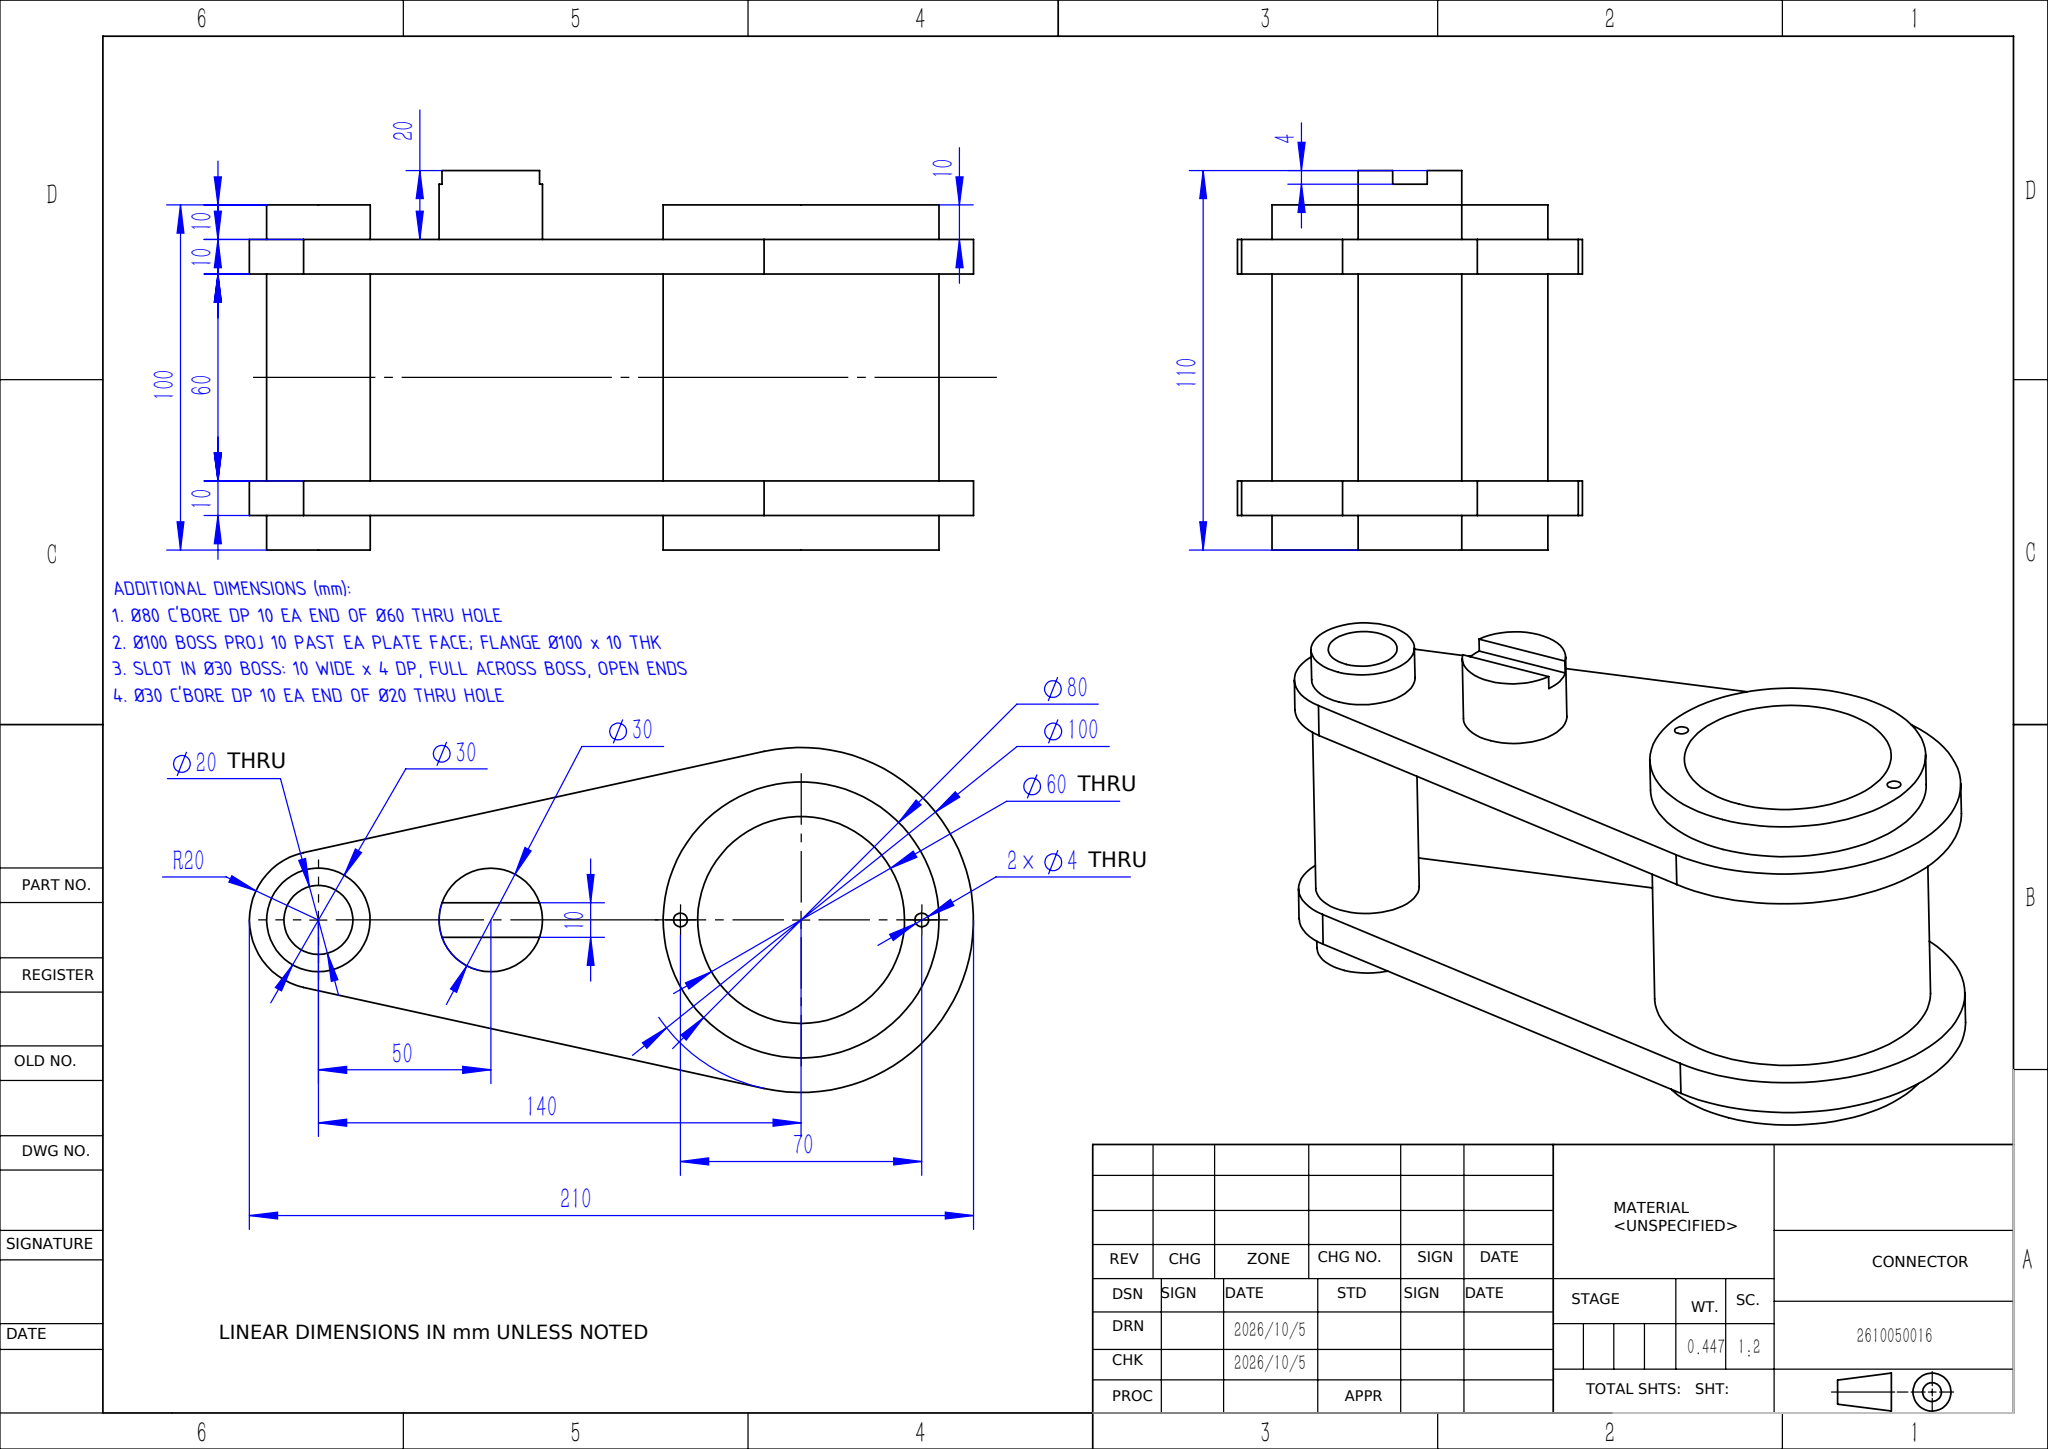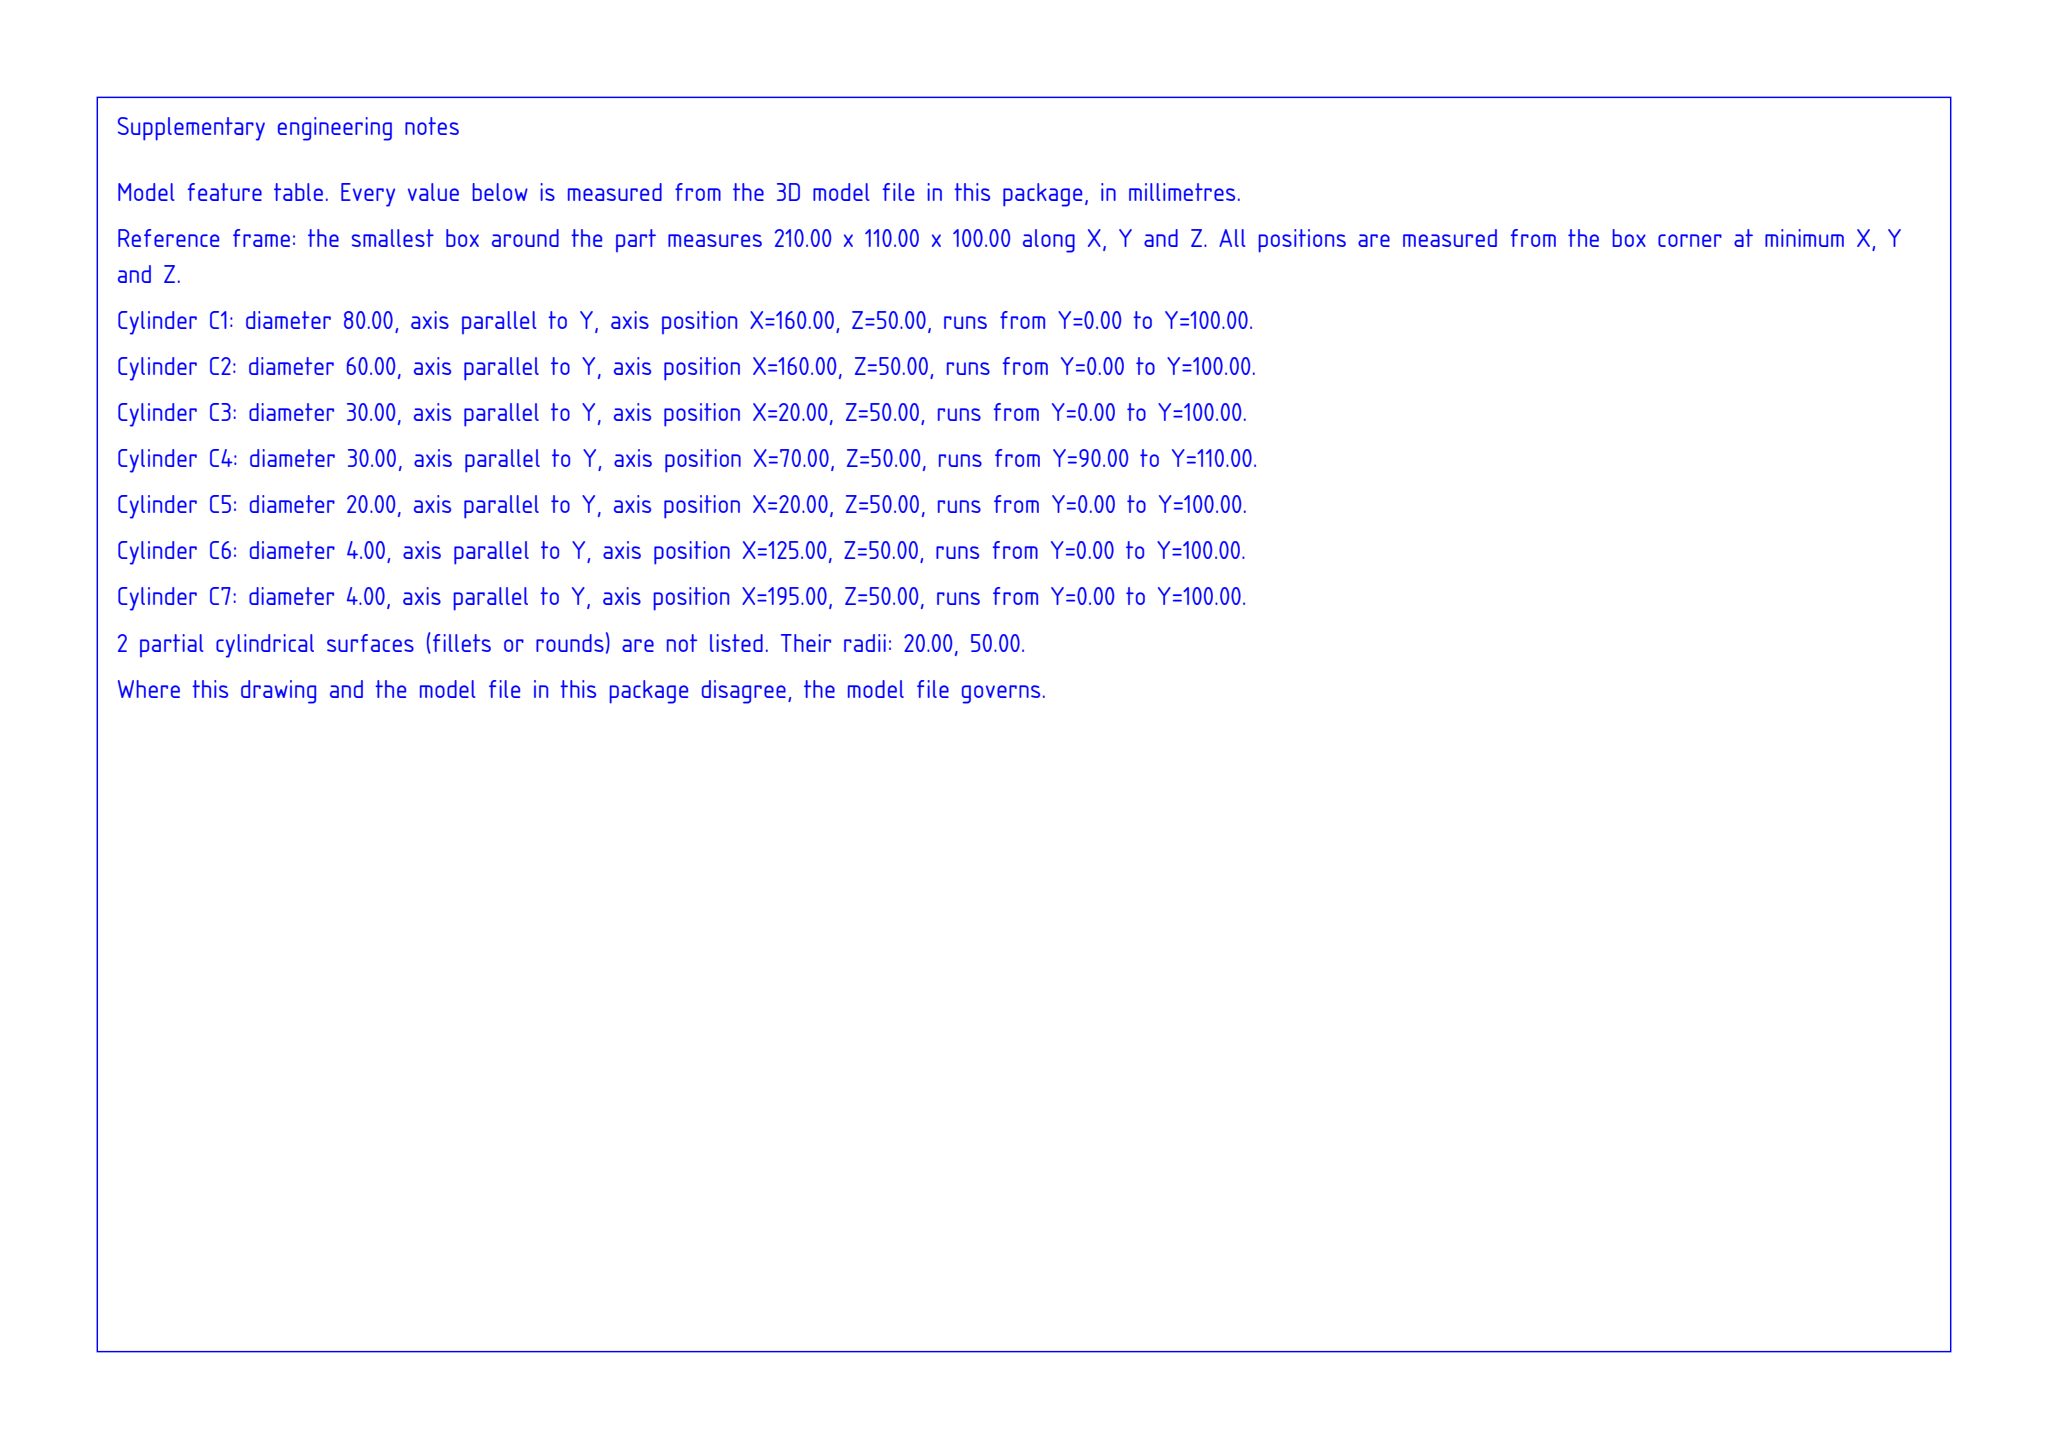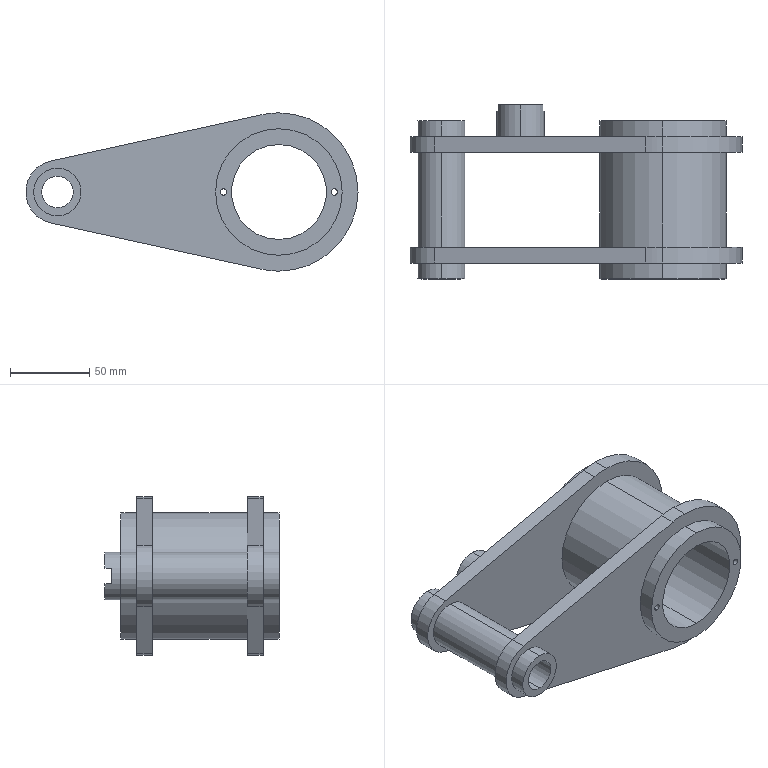Part | SolidWorks | mm | 1 solid | 47 faces | box 210 x 110 x 100 mm | volume 446583 mm3 | cylinder 30 | plane 17 | commonest cylinder face diameters 30 x8 80 x6 100 x6 4 x4 20 x2 60 x2 40 x2
build123d program:
from build123d import *

# Parameters (mm, degrees)
BOSS_EXTRUDE1_DEPTH     = 40
CUT_EXTRUDE1_DEPTH      = 137.015
CUT_EXTRUDE1_DEPTH_BACK = 137.015
SKETCH2_W               = 210
SKETCH2_H               = 60
SKETCH3_R               = 15
SKETCH3_R_2             = 40
BOSS_EXTRUDE2_DEPTH     = 50
CUT_EXTRUDE2_DEPTH      = 165.012
CUT_EXTRUDE2_DEPTH_BACK = 165.012
SKETCH4_R               = 10
SKETCH4_R_2             = 30
SKETCH5_R               = 15
BOSS_EXTRUDE3_DEPTH     = 20
CUT_EXTRUDE3_DEPTH      = 171.294
CUT_EXTRUDE3_DEPTH_BACK = 4
SKETCH6_W               = 33.027
SKETCH6_H               = 10
SKETCH7_R               = 2
CUT_EXTRUDE4_DEPTH      = 165.012


with BuildPart() as part:
    # Sketch1 → Boss-Extrude1 (new, symmetric)
    with BuildSketch(Plane(origin=(0, 0, 0), x_dir=(1, 0, 0), z_dir=(0, 1, 0))):
        with BuildLine():
            Line((-74.286, 19.535), (59.286, 48.839))
            ThreePointArc((59.286, 48.839), (120, 0), (59.286, -48.839))
            Line((59.286, -48.839), (-74.286, -19.535))
            ThreePointArc((-74.286, -19.535), (-90, 0), (-74.286, 19.535))
        make_face()
    extrude(amount=BOSS_EXTRUDE1_DEPTH, both=True)

    # Sketch2 → Cut-Extrude1 (cut, two sides: drawn at the far end of the back side and taken through both)
    with BuildSketch(Plane.XY.offset(-CUT_EXTRUDE1_DEPTH_BACK)):
        with Locations((15, 0)):
            Rectangle(SKETCH2_W, SKETCH2_H)
    extrude(amount=CUT_EXTRUDE1_DEPTH + CUT_EXTRUDE1_DEPTH_BACK, mode=Mode.SUBTRACT)


with BuildPart() as cut_extrude1_piece_1:
    # of the separate pieces the step leaves, piece 1, a body of its own (cut_extrude1_pieces)
    add(part.part.solids().sort_by_distance((59.286, 30, 48.839))[0])



with BuildPart() as cut_extrude1_piece_2:
    # of the separate pieces the step leaves, piece 2, a body of its own (cut_extrude1_pieces)
    add(part.part.solids().sort_by_distance((59.286, -40, 48.839))[0])


with BuildPart() as cut_extrude1_piece_1_1:
    add(cut_extrude1_piece_1.part)

    add(cut_extrude1_piece_2.part)  # Boss-Extrude2 merges Cut-Extrude1 piece 2
    # Sketch3 → Boss-Extrude2 (add, symmetric)
    with BuildSketch(Plane(origin=(0, 0, 0), x_dir=(1, 0, 0), z_dir=(0, 1, 0))):
        with Locations(Location((-70, 0, 0), (0, 0, 90))):
            Circle(SKETCH3_R)
        with Locations(Location((70, 0, 0), (0, 0, 90))):
            Circle(SKETCH3_R_2)
    extrude(amount=BOSS_EXTRUDE2_DEPTH, both=True)

    # Sketch4 → Cut-Extrude2 (cut, two sides: drawn at the far end of the back side and taken through both)
    with BuildSketch(Plane(origin=(0, 50, 0), x_dir=(1, 0, 0), z_dir=(0, 1, 0)).offset(-CUT_EXTRUDE2_DEPTH_BACK)):
        with Locations(Location((-70, 0, 0), (0, 0, 270))):
            Circle(SKETCH4_R)
        with Locations(Location((70, 0, 0), (0, 0, 270))):
            Circle(SKETCH4_R_2)
    extrude(amount=CUT_EXTRUDE2_DEPTH + CUT_EXTRUDE2_DEPTH_BACK, mode=Mode.SUBTRACT)

    # Sketch5 → Boss-Extrude3 (add)
    with BuildSketch(Plane(origin=(0, 40, 0), x_dir=(1, 0, 0), z_dir=(0, 1, 0))):
        with Locations(Location((-20, 0, 0), (0, 0, 270))):
            Circle(SKETCH5_R)
    extrude(amount=BOSS_EXTRUDE3_DEPTH)

    # Sketch6 → Cut-Extrude3 (cut, two sides: drawn at the far end of the back side and taken through both)
    with BuildSketch(Plane(origin=(0, 60, 0), x_dir=(1, 0, 0), z_dir=(0, 1, 0)).offset(-CUT_EXTRUDE3_DEPTH_BACK)):
        with Locations((-19.876, 0)):
            Rectangle(SKETCH6_W, SKETCH6_H)
    extrude(amount=CUT_EXTRUDE3_DEPTH + CUT_EXTRUDE3_DEPTH_BACK, mode=Mode.SUBTRACT)

    # Sketch7 → Cut-Extrude4 (cut, through all)
    with BuildSketch(Plane(origin=(0, 50, 0), x_dir=(1, 0, 0), z_dir=(0, 1, 0))):
        with Locations(Location((35, 0, 0), (0, 0, 270))):
            Circle(SKETCH7_R)
        with Locations(Location((105, 0, 0), (0, 0, 270))):
            Circle(SKETCH7_R)
    extrude(amount=-CUT_EXTRUDE4_DEPTH, mode=Mode.SUBTRACT)


solid = cut_extrude1_piece_1_1.part